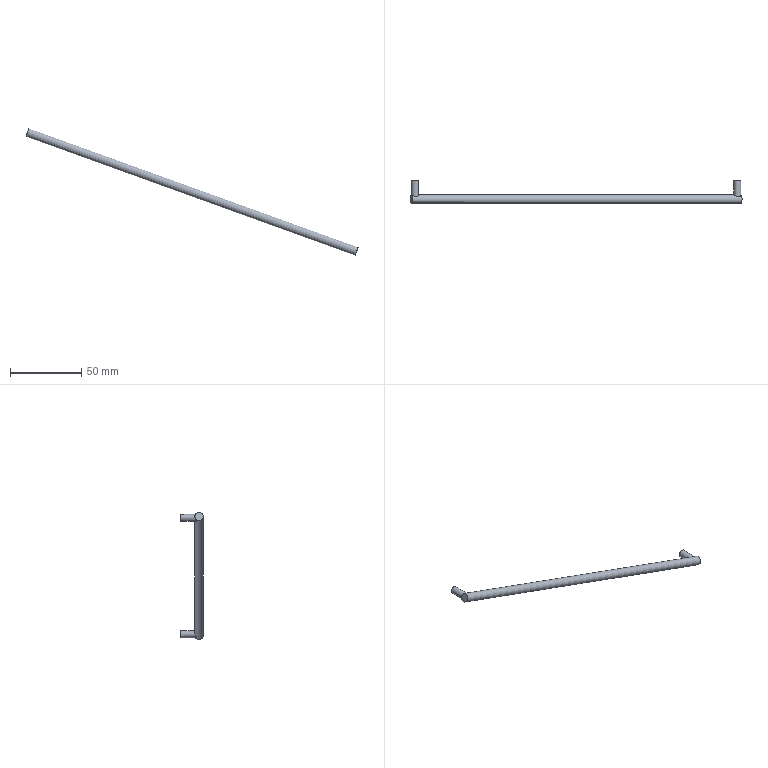Component | NX | LINK_2 | 1 solid | 7 faces | volume 7331 mm3 | plane 4 | cylinder 3 | commonest cylinder face diameters 5 x2 6 x1